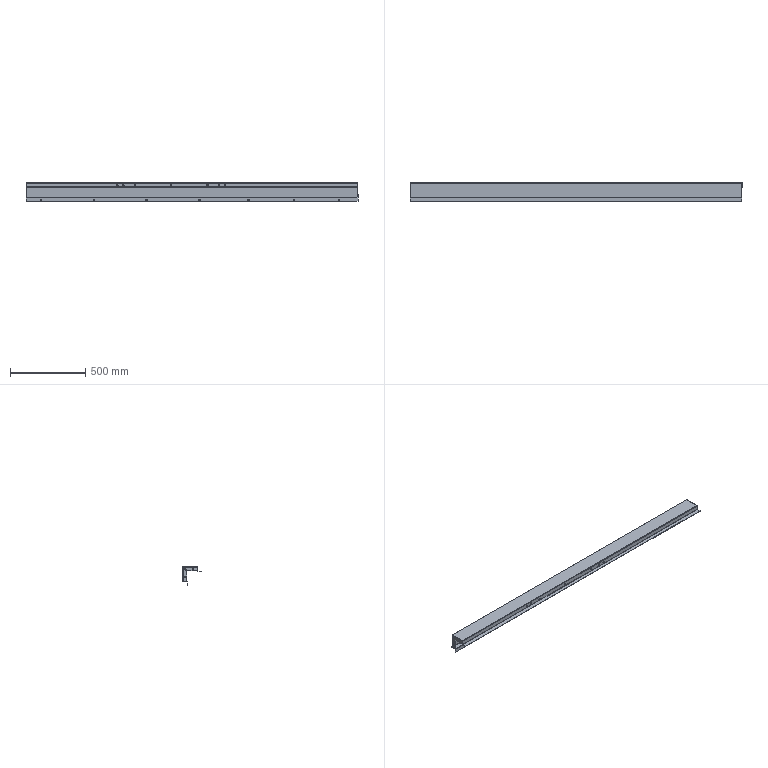Component | SolidWorks | 13FrontUpperBeam-1 | 1 solid | 144 faces | volume 1348257 mm3 | cylinder 76 | plane 64 | spline 4 | commonest cylinder face diameters 10 x58 6 x9 2 x9